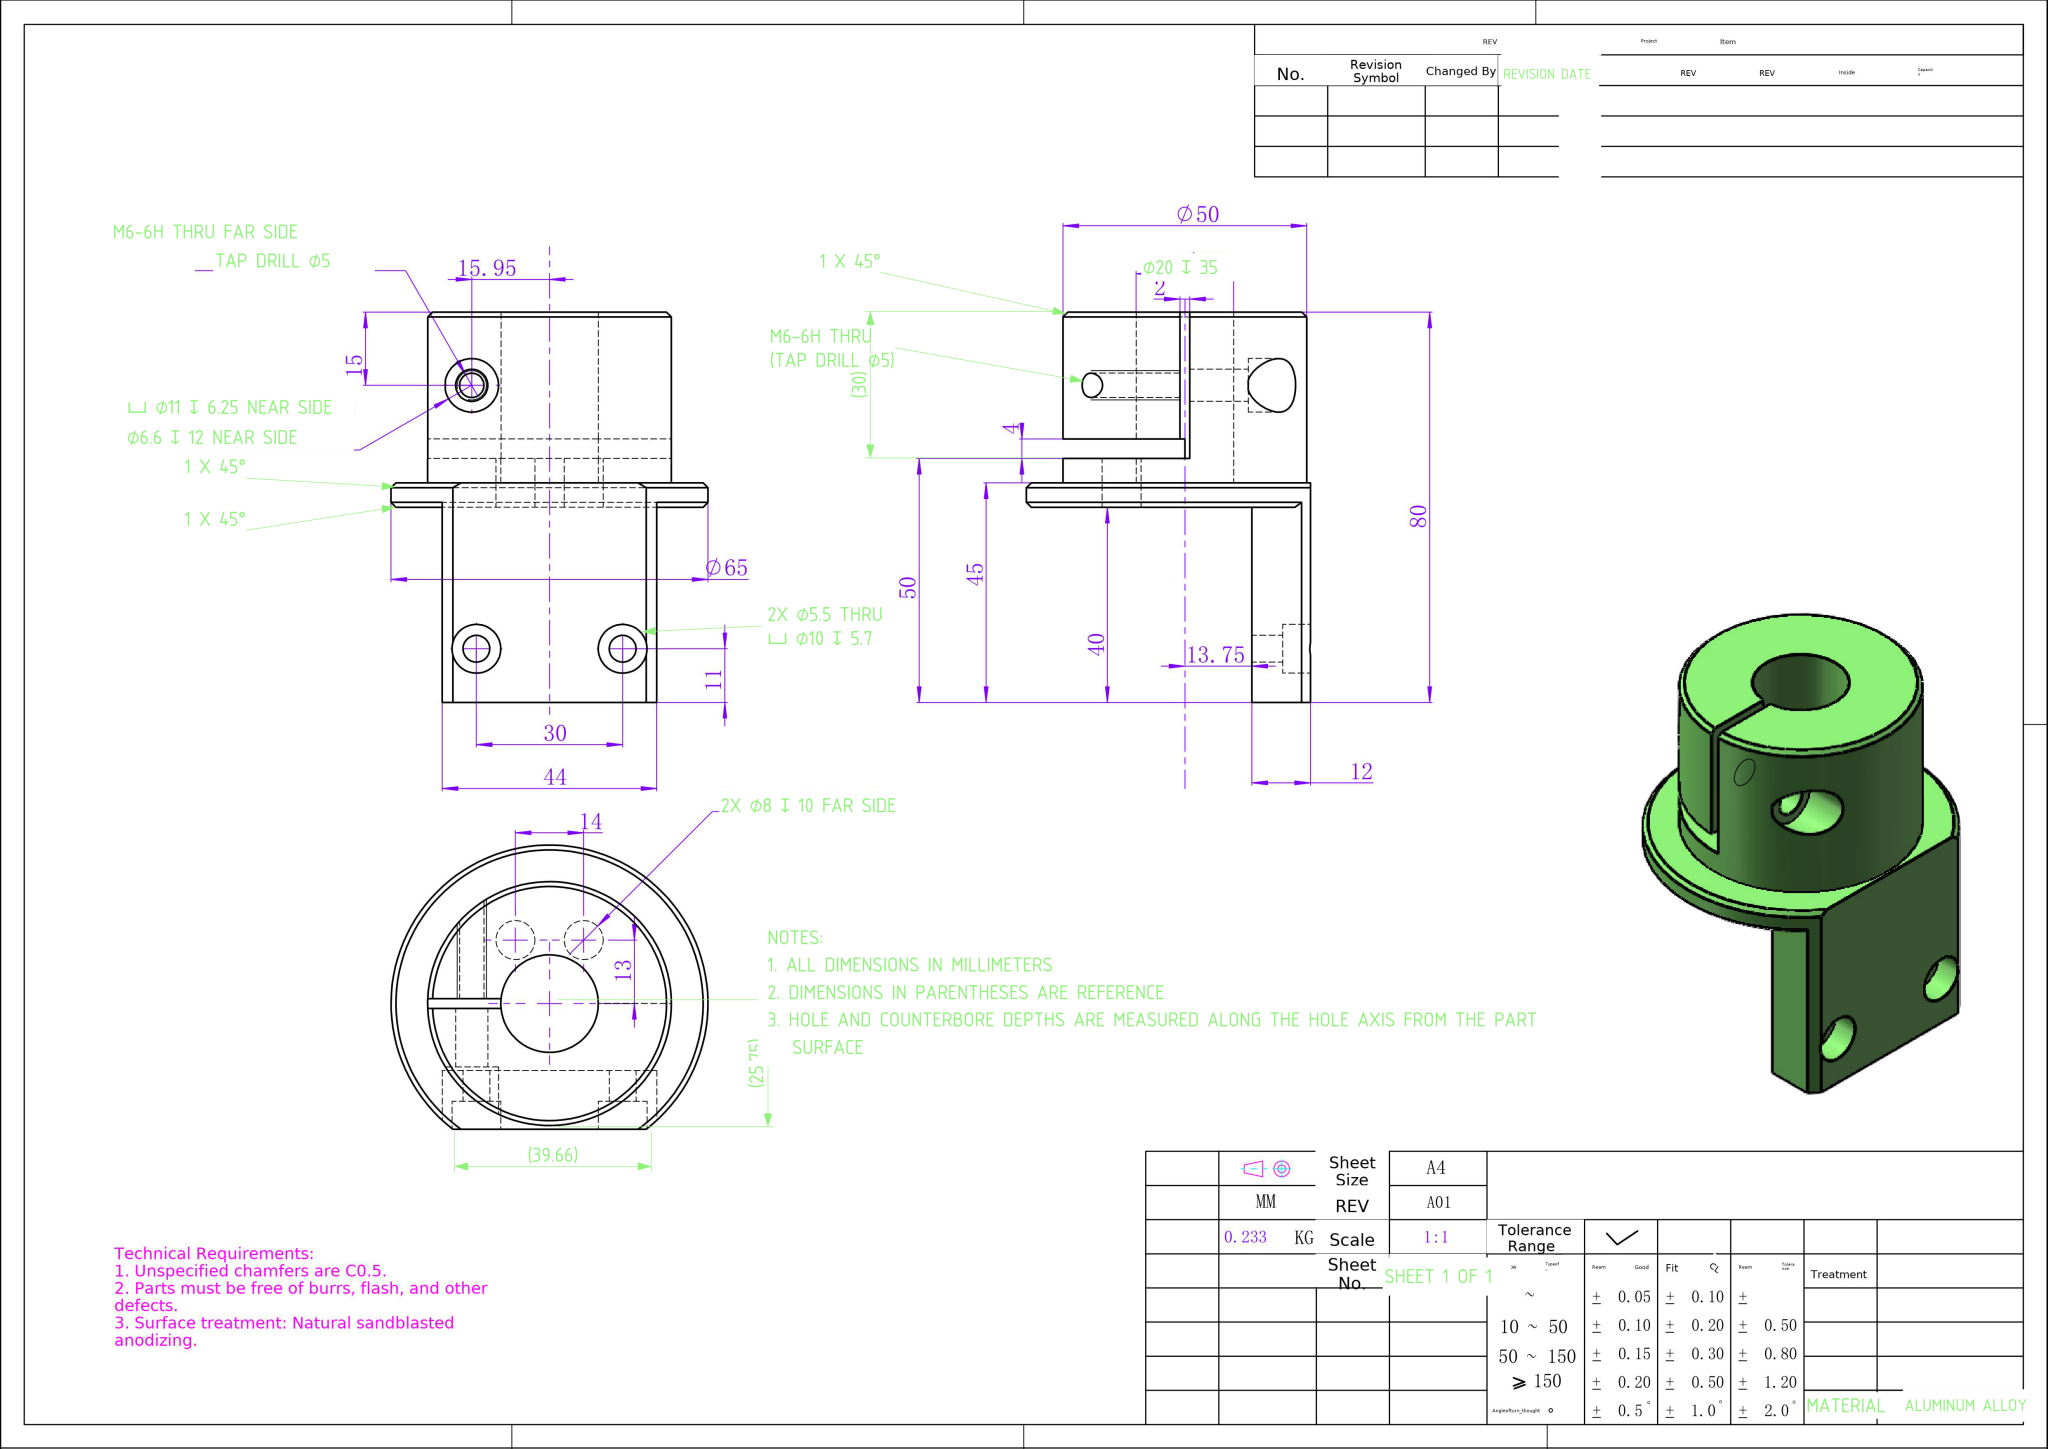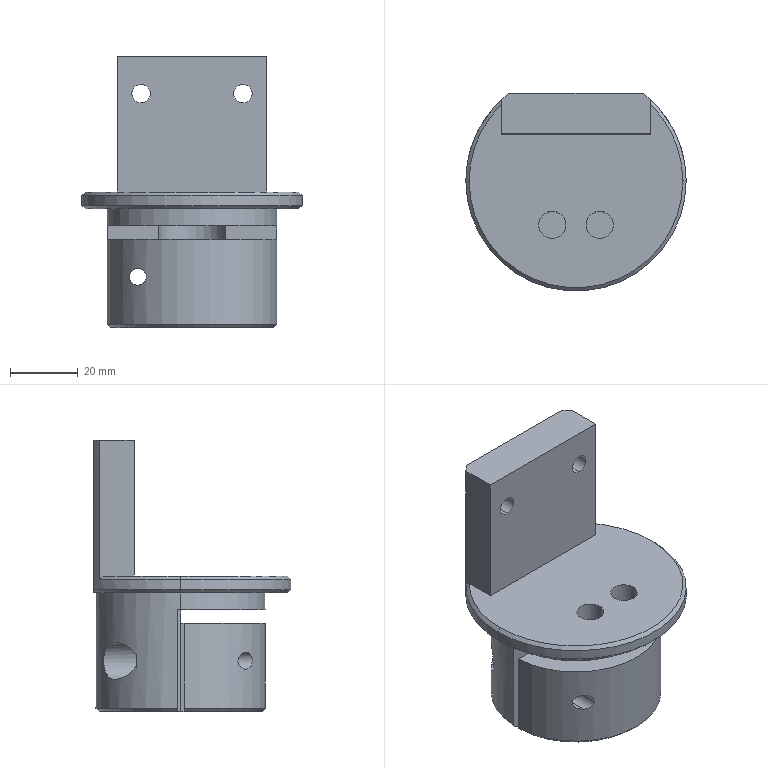Part | NX | mm | 1 solid | 53 faces | box 65 x 58.25 x 80 mm | volume 86470 mm3 | cylinder 28 | plane 17 | cone 8 | commonest cylinder face diameters 8 x4 5.5 x4 10 x4 11 x3 20 x3 65 x3 50 x3 5 x2